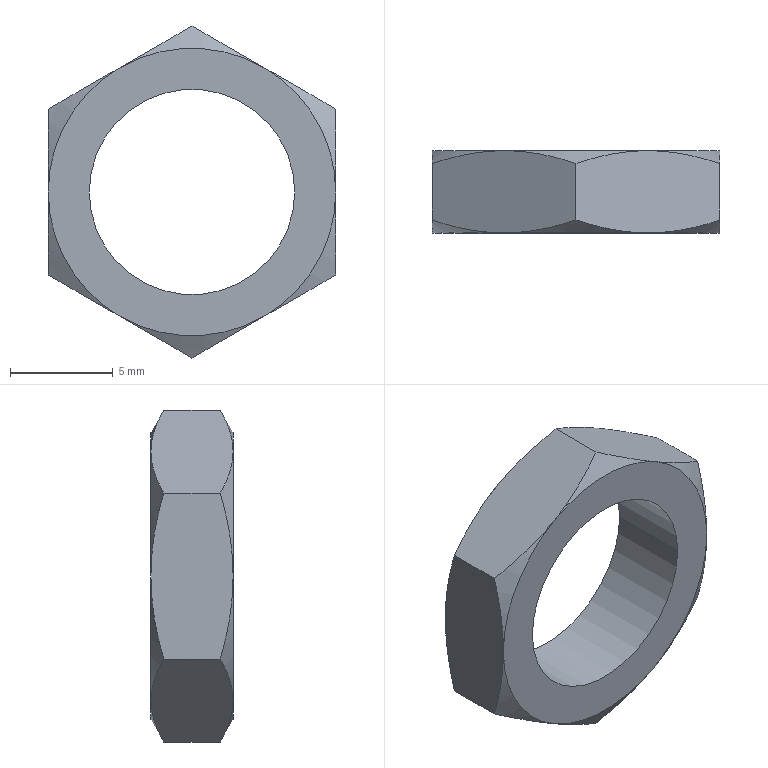Component | SolidWorks | ClampingAssembly-1_RB1006-1_RB1006-2-1 | 1 solid | 22 faces | box 14 x 4 x 16.17 mm | volume 359 mm3 | cone 12 | plane 8 | cylinder 2 | commonest cylinder face diameters 10 x2
STEP:
#1=COLOUR_RGB('',0.7922,0.8196,0.9333);
#2=FILL_AREA_STYLE_COLOUR('',#1);
#3=FILL_AREA_STYLE('',(#2));
#4=SURFACE_STYLE_FILL_AREA(#3);
#5=SURFACE_SIDE_STYLE('',(#4));
#6=SURFACE_STYLE_USAGE(.BOTH.,#5);
#7=PRESENTATION_STYLE_ASSIGNMENT((#6));
#8=CARTESIAN_POINT('',(-0.1398,4.726,-1.201));
#9=VERTEX_POINT('',#8);
#10=CARTESIAN_POINT('',(-0.5335,4.726,-1.201));
#11=VERTEX_POINT('',#10);
#12=CARTESIAN_POINT('',(-0.3366,4.726,-1.201));
#13=DIRECTION('',(-0.,1.,-0.));
#14=DIRECTION('',(-1.,0.,0.));
#15=AXIS2_PLACEMENT_3D('',#12,#13,#14);
#16=CIRCLE('',#15,0.1969);
#17=EDGE_CURVE('',#9,#11,#16,.T.);
#18=ORIENTED_EDGE('',*,*,#17,.T.);
#19=CARTESIAN_POINT('',(-0.5335,4.568,-1.201));
#20=VERTEX_POINT('',#19);
#21=CARTESIAN_POINT('',(-0.5335,4.568,-1.201));
#22=DIRECTION('',(0.,-1.,0.));
#23=VECTOR('',#22,39.37);
#24=LINE('',#21,#23);
#25=EDGE_CURVE('',#11,#20,#24,.T.);
#26=ORIENTED_EDGE('',*,*,#25,.T.);
#27=CARTESIAN_POINT('',(-0.1398,4.568,-1.201));
#28=VERTEX_POINT('',#27);
#29=CARTESIAN_POINT('',(-0.3366,4.568,-1.201));
#30=DIRECTION('',(-0.,1.,-0.));
#31=DIRECTION('',(1.,0.,0.));
#32=AXIS2_PLACEMENT_3D('',#29,#30,#31);
#33=CIRCLE('',#32,0.1969);
#34=EDGE_CURVE('',#28,#20,#33,.T.);
#35=ORIENTED_EDGE('',*,*,#34,.F.);
#36=CARTESIAN_POINT('',(-0.1398,4.568,-1.201));
#37=DIRECTION('',(0.,-1.,0.));
#38=VECTOR('',#37,39.37);
#39=LINE('',#36,#38);
#40=EDGE_CURVE('',#9,#28,#39,.T.);
#41=ORIENTED_EDGE('',*,*,#40,.F.);
#42=EDGE_LOOP('',(#18,#26,#35,#41));
#43=FACE_OUTER_BOUND('',#42,.T.);
#44=CARTESIAN_POINT('',(-0.3366,4.568,-1.201));
#45=DIRECTION('',(0.,-1.,0.));
#46=DIRECTION('',(1.,0.,0.));
#47=AXIS2_PLACEMENT_3D('',#44,#45,#46);
#48=CYLINDRICAL_SURFACE('',#47,0.1969);
#49=ADVANCED_FACE('',(#43),#48,.F.);
#50=CARTESIAN_POINT('',(-0.1988,4.568,-1.439));
#51=VERTEX_POINT('',#50);
#52=CARTESIAN_POINT('',(-0.06105,4.568,-1.201));
#53=VERTEX_POINT('',#52);
#54=CARTESIAN_POINT('',(-0.3366,4.568,-1.201));
#55=DIRECTION('',(-0.,-1.,0.));
#56=DIRECTION('',(-1.,0.,0.));
#57=AXIS2_PLACEMENT_3D('',#54,#55,#56);
#58=CIRCLE('',#57,0.2756);
#59=EDGE_CURVE('',#51,#53,#58,.T.);
#60=ORIENTED_EDGE('',*,*,#59,.T.);
#61=CARTESIAN_POINT('',(-0.1988,4.568,-0.9621));
#62=VERTEX_POINT('',#61);
#63=CARTESIAN_POINT('',(-0.3366,4.568,-1.201));
#64=DIRECTION('',(-0.,-1.,0.));
#65=DIRECTION('',(-1.,0.,0.));
#66=AXIS2_PLACEMENT_3D('',#63,#64,#65);
#67=CIRCLE('',#66,0.2756);
#68=EDGE_CURVE('',#53,#62,#67,.T.);
#69=ORIENTED_EDGE('',*,*,#68,.T.);
#70=CARTESIAN_POINT('',(-0.4744,4.568,-0.9621));
#71=VERTEX_POINT('',#70);
#72=CARTESIAN_POINT('',(-0.3366,4.568,-1.201));
#73=DIRECTION('',(0.,-1.,0.));
#74=DIRECTION('',(-1.,0.,0.));
#75=AXIS2_PLACEMENT_3D('',#72,#73,#74);
#76=CIRCLE('',#75,0.2756);
#77=EDGE_CURVE('',#62,#71,#76,.T.);
#78=ORIENTED_EDGE('',*,*,#77,.T.);
#79=CARTESIAN_POINT('',(-0.6122,4.568,-1.201));
#80=VERTEX_POINT('',#79);
#81=CARTESIAN_POINT('',(-0.3366,4.568,-1.201));
#82=DIRECTION('',(-0.,-1.,0.));
#83=DIRECTION('',(-1.,0.,0.));
#84=AXIS2_PLACEMENT_3D('',#81,#82,#83);
#85=CIRCLE('',#84,0.2756);
#86=EDGE_CURVE('',#71,#80,#85,.T.);
#87=ORIENTED_EDGE('',*,*,#86,.T.);
#88=CARTESIAN_POINT('',(-0.4744,4.568,-1.439));
#89=VERTEX_POINT('',#88);
#90=CARTESIAN_POINT('',(-0.3366,4.568,-1.201));
#91=DIRECTION('',(-0.,-1.,0.));
#92=DIRECTION('',(-1.,0.,-0.));
#93=AXIS2_PLACEMENT_3D('',#90,#91,#92);
#94=CIRCLE('',#93,0.2756);
#95=EDGE_CURVE('',#80,#89,#94,.T.);
#96=ORIENTED_EDGE('',*,*,#95,.T.);
#97=CARTESIAN_POINT('',(-0.3366,4.568,-1.201));
#98=DIRECTION('',(0.,-1.,0.));
#99=DIRECTION('',(-1.,0.,0.));
#100=AXIS2_PLACEMENT_3D('',#97,#98,#99);
#101=CIRCLE('',#100,0.2756);
#102=EDGE_CURVE('',#89,#51,#101,.T.);
#103=ORIENTED_EDGE('',*,*,#102,.T.);
#104=EDGE_LOOP('',(#60,#69,#78,#87,#96,#103));
#105=FACE_OUTER_BOUND('',#104,.T.);
#106=ORIENTED_EDGE('',*,*,#34,.T.);
#107=CARTESIAN_POINT('',(-0.3366,4.568,-1.201));
#108=DIRECTION('',(-0.,1.,-0.));
#109=DIRECTION('',(1.,0.,0.));
#110=AXIS2_PLACEMENT_3D('',#107,#108,#109);
#111=CIRCLE('',#110,0.1969);
#112=EDGE_CURVE('',#20,#28,#111,.T.);
#113=ORIENTED_EDGE('',*,*,#112,.T.);
#114=EDGE_LOOP('',(#106,#113));
#115=FACE_BOUND('',#114,.T.);
#116=CARTESIAN_POINT('',(-0.3366,4.568,-0.9646));
#117=DIRECTION('',(0.,-1.,0.));
#118=DIRECTION('',(1.,0.,-0.));
#119=AXIS2_PLACEMENT_3D('',#116,#117,#118);
#120=PLANE('',#119);
#121=ADVANCED_FACE('',(#105,#115),#120,.T.);
#122=CARTESIAN_POINT('',(-0.06105,4.593,-1.042));
#123=VERTEX_POINT('',#122);
#124=CARTESIAN_POINT('',(-0.06105,4.593,-1.042));
#125=CARTESIAN_POINT('',(-0.08356,4.585,-1.029));
#126=CARTESIAN_POINT('',(-0.1063,4.579,-1.016));
#127=CARTESIAN_POINT('',(-0.1521,4.571,-0.9891));
#128=CARTESIAN_POINT('',(-0.1753,4.568,-0.9757));
#129=CARTESIAN_POINT('',(-0.1988,4.568,-0.9621));
#130=B_SPLINE_CURVE_WITH_KNOTS('',3,(#124,#125,#126,#127,#128,#129),.UNSPECIFIED.,.F.,.F.,(4,2,4),(0.,0.002045,0.00409),.UNSPECIFIED.);
#131=EDGE_CURVE('',#123,#62,#130,.T.);
#132=ORIENTED_EDGE('',*,*,#131,.T.);
#133=ORIENTED_EDGE('',*,*,#68,.F.);
#134=CARTESIAN_POINT('',(-0.06105,4.568,-1.201));
#135=CARTESIAN_POINT('',(-0.06105,4.568,-1.174));
#136=CARTESIAN_POINT('',(-0.06105,4.571,-1.147));
#137=CARTESIAN_POINT('',(-0.06105,4.579,-1.094));
#138=CARTESIAN_POINT('',(-0.06105,4.585,-1.068));
#139=CARTESIAN_POINT('',(-0.06105,4.593,-1.042));
#140=B_SPLINE_CURVE_WITH_KNOTS('',3,(#134,#135,#136,#137,#138,#139),.UNSPECIFIED.,.F.,.F.,(4,2,4),(0.,0.002045,0.00409),.UNSPECIFIED.);
#141=EDGE_CURVE('',#53,#123,#140,.T.);
#142=ORIENTED_EDGE('',*,*,#141,.T.);
#143=EDGE_LOOP('',(#132,#133,#142));
#144=FACE_OUTER_BOUND('',#143,.T.);
#145=CARTESIAN_POINT('',(-0.3366,4.593,-1.201));
#146=DIRECTION('',(0.,1.,-0.));
#147=DIRECTION('',(-1.,0.,0.));
#148=AXIS2_PLACEMENT_3D('',#145,#146,#147);
#149=CONICAL_SURFACE('',#148,0.3185,1.047);
#150=ADVANCED_FACE('',(#144),#149,.T.);
#151=CARTESIAN_POINT('',(-0.06105,4.593,-1.36));
#152=VERTEX_POINT('',#151);
#153=CARTESIAN_POINT('',(-0.06105,4.593,-1.36));
#154=CARTESIAN_POINT('',(-0.06105,4.585,-1.334));
#155=CARTESIAN_POINT('',(-0.06105,4.579,-1.308));
#156=CARTESIAN_POINT('',(-0.06105,4.571,-1.255));
#157=CARTESIAN_POINT('',(-0.06105,4.568,-1.228));
#158=CARTESIAN_POINT('',(-0.06105,4.568,-1.201));
#159=B_SPLINE_CURVE_WITH_KNOTS('',3,(#153,#154,#155,#156,#157,#158),.UNSPECIFIED.,.F.,.F.,(4,2,4),(0.,0.002045,0.00409),.UNSPECIFIED.);
#160=EDGE_CURVE('',#152,#53,#159,.T.);
#161=ORIENTED_EDGE('',*,*,#160,.T.);
#162=ORIENTED_EDGE('',*,*,#59,.F.);
#163=CARTESIAN_POINT('',(-0.1988,4.568,-1.439));
#164=CARTESIAN_POINT('',(-0.1753,4.568,-1.426));
#165=CARTESIAN_POINT('',(-0.1521,4.571,-1.412));
#166=CARTESIAN_POINT('',(-0.1063,4.579,-1.386));
#167=CARTESIAN_POINT('',(-0.08356,4.585,-1.373));
#168=CARTESIAN_POINT('',(-0.06105,4.593,-1.36));
#169=B_SPLINE_CURVE_WITH_KNOTS('',3,(#163,#164,#165,#166,#167,#168),.UNSPECIFIED.,.F.,.F.,(4,2,4),(0.,0.002045,0.00409),.UNSPECIFIED.);
#170=EDGE_CURVE('',#51,#152,#169,.T.);
#171=ORIENTED_EDGE('',*,*,#170,.T.);
#172=EDGE_LOOP('',(#161,#162,#171));
#173=FACE_OUTER_BOUND('',#172,.T.);
#174=CARTESIAN_POINT('',(-0.3366,4.593,-1.201));
#175=DIRECTION('',(0.,1.,-0.));
#176=DIRECTION('',(-1.,0.,0.));
#177=AXIS2_PLACEMENT_3D('',#174,#175,#176);
#178=CONICAL_SURFACE('',#177,0.3185,1.047);
#179=ADVANCED_FACE('',(#173),#178,.T.);
#180=CARTESIAN_POINT('',(-0.3366,4.593,-1.519));
#181=VERTEX_POINT('',#180);
#182=CARTESIAN_POINT('',(-0.3366,4.593,-1.519));
#183=CARTESIAN_POINT('',(-0.3141,4.585,-1.506));
#184=CARTESIAN_POINT('',(-0.2914,4.579,-1.493));
#185=CARTESIAN_POINT('',(-0.2456,4.571,-1.466));
#186=CARTESIAN_POINT('',(-0.2224,4.568,-1.453));
#187=CARTESIAN_POINT('',(-0.1988,4.568,-1.439));
#188=B_SPLINE_CURVE_WITH_KNOTS('',3,(#182,#183,#184,#185,#186,#187),.UNSPECIFIED.,.F.,.F.,(4,2,4),(0.,0.002045,0.00409),.UNSPECIFIED.);
#189=EDGE_CURVE('',#181,#51,#188,.T.);
#190=ORIENTED_EDGE('',*,*,#189,.T.);
#191=ORIENTED_EDGE('',*,*,#102,.F.);
#192=CARTESIAN_POINT('',(-0.4744,4.568,-1.439));
#193=CARTESIAN_POINT('',(-0.4509,4.568,-1.453));
#194=CARTESIAN_POINT('',(-0.4277,4.571,-1.466));
#195=CARTESIAN_POINT('',(-0.3818,4.579,-1.493));
#196=CARTESIAN_POINT('',(-0.3592,4.585,-1.506));
#197=CARTESIAN_POINT('',(-0.3366,4.593,-1.519));
#198=B_SPLINE_CURVE_WITH_KNOTS('',3,(#192,#193,#194,#195,#196,#197),.UNSPECIFIED.,.F.,.F.,(4,2,4),(0.,0.002045,0.00409),.UNSPECIFIED.);
#199=EDGE_CURVE('',#89,#181,#198,.T.);
#200=ORIENTED_EDGE('',*,*,#199,.T.);
#201=EDGE_LOOP('',(#190,#191,#200));
#202=FACE_OUTER_BOUND('',#201,.T.);
#203=CARTESIAN_POINT('',(-0.3366,4.593,-1.201));
#204=DIRECTION('',(-0.,1.,-0.));
#205=DIRECTION('',(-1.,0.,0.));
#206=AXIS2_PLACEMENT_3D('',#203,#204,#205);
#207=CONICAL_SURFACE('',#206,0.3185,1.047);
#208=ADVANCED_FACE('',(#202),#207,.T.);
#209=ORIENTED_EDGE('',*,*,#95,.F.);
#210=CARTESIAN_POINT('',(-0.6122,4.593,-1.36));
#211=VERTEX_POINT('',#210);
#212=CARTESIAN_POINT('',(-0.6122,4.568,-1.201));
#213=CARTESIAN_POINT('',(-0.6122,4.568,-1.228));
#214=CARTESIAN_POINT('',(-0.6122,4.571,-1.255));
#215=CARTESIAN_POINT('',(-0.6122,4.579,-1.308));
#216=CARTESIAN_POINT('',(-0.6122,4.585,-1.334));
#217=CARTESIAN_POINT('',(-0.6122,4.593,-1.36));
#218=B_SPLINE_CURVE_WITH_KNOTS('',3,(#212,#213,#214,#215,#216,#217),.UNSPECIFIED.,.F.,.F.,(4,2,4),(0.,0.002045,0.00409),.UNSPECIFIED.);
#219=EDGE_CURVE('',#80,#211,#218,.T.);
#220=ORIENTED_EDGE('',*,*,#219,.T.);
#221=CARTESIAN_POINT('',(-0.6122,4.593,-1.36));
#222=CARTESIAN_POINT('',(-0.5897,4.585,-1.373));
#223=CARTESIAN_POINT('',(-0.567,4.579,-1.386));
#224=CARTESIAN_POINT('',(-0.5212,4.571,-1.412));
#225=CARTESIAN_POINT('',(-0.498,4.568,-1.426));
#226=CARTESIAN_POINT('',(-0.4744,4.568,-1.439));
#227=B_SPLINE_CURVE_WITH_KNOTS('',3,(#221,#222,#223,#224,#225,#226),.UNSPECIFIED.,.F.,.F.,(4,2,4),(0.,0.002045,0.00409),.UNSPECIFIED.);
#228=EDGE_CURVE('',#211,#89,#227,.T.);
#229=ORIENTED_EDGE('',*,*,#228,.T.);
#230=EDGE_LOOP('',(#209,#220,#229));
#231=FACE_OUTER_BOUND('',#230,.T.);
#232=CARTESIAN_POINT('',(-0.3366,4.593,-1.201));
#233=DIRECTION('',(0.,1.,-0.));
#234=DIRECTION('',(-1.,0.,0.));
#235=AXIS2_PLACEMENT_3D('',#232,#233,#234);
#236=CONICAL_SURFACE('',#235,0.3185,1.047);
#237=ADVANCED_FACE('',(#231),#236,.T.);
#238=ORIENTED_EDGE('',*,*,#86,.F.);
#239=CARTESIAN_POINT('',(-0.6122,4.593,-1.042));
#240=VERTEX_POINT('',#239);
#241=CARTESIAN_POINT('',(-0.4744,4.568,-0.9621));
#242=CARTESIAN_POINT('',(-0.498,4.568,-0.9757));
#243=CARTESIAN_POINT('',(-0.5212,4.571,-0.9891));
#244=CARTESIAN_POINT('',(-0.567,4.579,-1.016));
#245=CARTESIAN_POINT('',(-0.5897,4.585,-1.029));
#246=CARTESIAN_POINT('',(-0.6122,4.593,-1.042));
#247=B_SPLINE_CURVE_WITH_KNOTS('',3,(#241,#242,#243,#244,#245,#246),.UNSPECIFIED.,.F.,.F.,(4,2,4),(0.,0.002045,0.00409),.UNSPECIFIED.);
#248=EDGE_CURVE('',#71,#240,#247,.T.);
#249=ORIENTED_EDGE('',*,*,#248,.T.);
#250=CARTESIAN_POINT('',(-0.6122,4.593,-1.042));
#251=CARTESIAN_POINT('',(-0.6122,4.585,-1.068));
#252=CARTESIAN_POINT('',(-0.6122,4.579,-1.094));
#253=CARTESIAN_POINT('',(-0.6122,4.571,-1.147));
#254=CARTESIAN_POINT('',(-0.6122,4.568,-1.174));
#255=CARTESIAN_POINT('',(-0.6122,4.568,-1.201));
#256=B_SPLINE_CURVE_WITH_KNOTS('',3,(#250,#251,#252,#253,#254,#255),.UNSPECIFIED.,.F.,.F.,(4,2,4),(0.,0.002045,0.00409),.UNSPECIFIED.);
#257=EDGE_CURVE('',#240,#80,#256,.T.);
#258=ORIENTED_EDGE('',*,*,#257,.T.);
#259=EDGE_LOOP('',(#238,#249,#258));
#260=FACE_OUTER_BOUND('',#259,.T.);
#261=CARTESIAN_POINT('',(-0.3366,4.593,-1.201));
#262=DIRECTION('',(0.,1.,-0.));
#263=DIRECTION('',(-1.,0.,0.));
#264=AXIS2_PLACEMENT_3D('',#261,#262,#263);
#265=CONICAL_SURFACE('',#264,0.3185,1.047);
#266=ADVANCED_FACE('',(#260),#265,.T.);
#267=CARTESIAN_POINT('',(-0.3366,4.593,-0.8826));
#268=VERTEX_POINT('',#267);
#269=CARTESIAN_POINT('',(-0.3366,4.593,-0.8826));
#270=CARTESIAN_POINT('',(-0.3592,4.585,-0.8956));
#271=CARTESIAN_POINT('',(-0.3818,4.579,-0.9087));
#272=CARTESIAN_POINT('',(-0.4277,4.571,-0.9351));
#273=CARTESIAN_POINT('',(-0.4509,4.568,-0.9485));
#274=CARTESIAN_POINT('',(-0.4744,4.568,-0.9621));
#275=B_SPLINE_CURVE_WITH_KNOTS('',3,(#269,#270,#271,#272,#273,#274),.UNSPECIFIED.,.F.,.F.,(4,2,4),(0.,0.002045,0.00409),.UNSPECIFIED.);
#276=EDGE_CURVE('',#268,#71,#275,.T.);
#277=ORIENTED_EDGE('',*,*,#276,.T.);
#278=ORIENTED_EDGE('',*,*,#77,.F.);
#279=CARTESIAN_POINT('',(-0.1988,4.568,-0.9621));
#280=CARTESIAN_POINT('',(-0.2224,4.568,-0.9485));
#281=CARTESIAN_POINT('',(-0.2456,4.571,-0.9351));
#282=CARTESIAN_POINT('',(-0.2914,4.579,-0.9087));
#283=CARTESIAN_POINT('',(-0.3141,4.585,-0.8956));
#284=CARTESIAN_POINT('',(-0.3366,4.593,-0.8826));
#285=B_SPLINE_CURVE_WITH_KNOTS('',3,(#279,#280,#281,#282,#283,#284),.UNSPECIFIED.,.F.,.F.,(4,2,4),(0.,0.002045,0.00409),.UNSPECIFIED.);
#286=EDGE_CURVE('',#62,#268,#285,.T.);
#287=ORIENTED_EDGE('',*,*,#286,.T.);
#288=EDGE_LOOP('',(#277,#278,#287));
#289=FACE_OUTER_BOUND('',#288,.T.);
#290=CARTESIAN_POINT('',(-0.3366,4.593,-1.201));
#291=DIRECTION('',(-0.,1.,-0.));
#292=DIRECTION('',(-1.,0.,0.));
#293=AXIS2_PLACEMENT_3D('',#290,#291,#292);
#294=CONICAL_SURFACE('',#293,0.3185,1.047);
#295=ADVANCED_FACE('',(#289),#294,.T.);
#296=CARTESIAN_POINT('',(-0.3366,4.701,-0.8826));
#297=VERTEX_POINT('',#296);
#298=CARTESIAN_POINT('',(-0.3366,4.568,-0.8826));
#299=DIRECTION('',(-0.,1.,-0.));
#300=VECTOR('',#299,39.37);
#301=LINE('',#298,#300);
#302=EDGE_CURVE('',#268,#297,#301,.T.);
#303=ORIENTED_EDGE('',*,*,#302,.F.);
#304=ORIENTED_EDGE('',*,*,#286,.F.);
#305=ORIENTED_EDGE('',*,*,#131,.F.);
#306=CARTESIAN_POINT('',(-0.06105,4.701,-1.042));
#307=VERTEX_POINT('',#306);
#308=CARTESIAN_POINT('',(-0.06105,4.568,-1.042));
#309=DIRECTION('',(0.,-1.,0.));
#310=VECTOR('',#309,39.37);
#311=LINE('',#308,#310);
#312=EDGE_CURVE('',#307,#123,#311,.T.);
#313=ORIENTED_EDGE('',*,*,#312,.F.);
#314=CARTESIAN_POINT('',(-0.1988,4.726,-0.9621));
#315=VERTEX_POINT('',#314);
#316=CARTESIAN_POINT('',(-0.1988,4.726,-0.9621));
#317=CARTESIAN_POINT('',(-0.1753,4.726,-0.9757));
#318=CARTESIAN_POINT('',(-0.1521,4.723,-0.9891));
#319=CARTESIAN_POINT('',(-0.1063,4.715,-1.016));
#320=CARTESIAN_POINT('',(-0.08356,4.709,-1.029));
#321=CARTESIAN_POINT('',(-0.06105,4.701,-1.042));
#322=B_SPLINE_CURVE_WITH_KNOTS('',3,(#316,#317,#318,#319,#320,#321),.UNSPECIFIED.,.F.,.F.,(4,2,4),(0.,0.002045,0.00409),.UNSPECIFIED.);
#323=EDGE_CURVE('',#315,#307,#322,.T.);
#324=ORIENTED_EDGE('',*,*,#323,.F.);
#325=CARTESIAN_POINT('',(-0.3366,4.701,-0.8826));
#326=CARTESIAN_POINT('',(-0.3141,4.709,-0.8956));
#327=CARTESIAN_POINT('',(-0.2914,4.715,-0.9087));
#328=CARTESIAN_POINT('',(-0.2456,4.723,-0.9351));
#329=CARTESIAN_POINT('',(-0.2224,4.726,-0.9485));
#330=CARTESIAN_POINT('',(-0.1988,4.726,-0.9621));
#331=B_SPLINE_CURVE_WITH_KNOTS('',3,(#325,#326,#327,#328,#329,#330),.UNSPECIFIED.,.F.,.F.,(4,2,4),(0.,0.002045,0.00409),.UNSPECIFIED.);
#332=EDGE_CURVE('',#297,#315,#331,.T.);
#333=ORIENTED_EDGE('',*,*,#332,.F.);
#334=EDGE_LOOP('',(#303,#304,#305,#313,#324,#333));
#335=FACE_OUTER_BOUND('',#334,.T.);
#336=CARTESIAN_POINT('',(-0.3366,4.568,-0.8826));
#337=DIRECTION('',(-0.5,-0.,-0.866));
#338=DIRECTION('',(-0.866,-0.,0.5));
#339=AXIS2_PLACEMENT_3D('',#336,#337,#338);
#340=PLANE('',#339);
#341=ADVANCED_FACE('',(#335),#340,.F.);
#342=CARTESIAN_POINT('',(-0.06105,4.726,-1.201));
#343=VERTEX_POINT('',#342);
#344=CARTESIAN_POINT('',(-0.06105,4.701,-1.042));
#345=CARTESIAN_POINT('',(-0.06105,4.709,-1.068));
#346=CARTESIAN_POINT('',(-0.06105,4.715,-1.094));
#347=CARTESIAN_POINT('',(-0.06105,4.723,-1.147));
#348=CARTESIAN_POINT('',(-0.06105,4.726,-1.174));
#349=CARTESIAN_POINT('',(-0.06105,4.726,-1.201));
#350=B_SPLINE_CURVE_WITH_KNOTS('',3,(#344,#345,#346,#347,#348,#349),.UNSPECIFIED.,.F.,.F.,(4,2,4),(0.,0.002045,0.00409),.UNSPECIFIED.);
#351=EDGE_CURVE('',#307,#343,#350,.T.);
#352=ORIENTED_EDGE('',*,*,#351,.F.);
#353=ORIENTED_EDGE('',*,*,#312,.T.);
#354=ORIENTED_EDGE('',*,*,#141,.F.);
#355=ORIENTED_EDGE('',*,*,#160,.F.);
#356=CARTESIAN_POINT('',(-0.06105,4.701,-1.36));
#357=VERTEX_POINT('',#356);
#358=CARTESIAN_POINT('',(-0.06105,4.568,-1.36));
#359=DIRECTION('',(0.,-1.,0.));
#360=VECTOR('',#359,39.37);
#361=LINE('',#358,#360);
#362=EDGE_CURVE('',#357,#152,#361,.T.);
#363=ORIENTED_EDGE('',*,*,#362,.F.);
#364=CARTESIAN_POINT('',(-0.06105,4.726,-1.201));
#365=CARTESIAN_POINT('',(-0.06105,4.726,-1.228));
#366=CARTESIAN_POINT('',(-0.06105,4.723,-1.255));
#367=CARTESIAN_POINT('',(-0.06105,4.715,-1.308));
#368=CARTESIAN_POINT('',(-0.06105,4.709,-1.334));
#369=CARTESIAN_POINT('',(-0.06105,4.701,-1.36));
#370=B_SPLINE_CURVE_WITH_KNOTS('',3,(#364,#365,#366,#367,#368,#369),.UNSPECIFIED.,.F.,.F.,(4,2,4),(0.,0.002045,0.00409),.UNSPECIFIED.);
#371=EDGE_CURVE('',#343,#357,#370,.T.);
#372=ORIENTED_EDGE('',*,*,#371,.F.);
#373=EDGE_LOOP('',(#352,#353,#354,#355,#363,#372));
#374=FACE_OUTER_BOUND('',#373,.T.);
#375=CARTESIAN_POINT('',(-0.06105,4.568,-1.042));
#376=DIRECTION('',(-1.,-0.,0.));
#377=DIRECTION('',(0.,-1.,0.));
#378=AXIS2_PLACEMENT_3D('',#375,#376,#377);
#379=PLANE('',#378);
#380=ADVANCED_FACE('',(#374),#379,.F.);
#381=CARTESIAN_POINT('',(-0.1988,4.726,-1.439));
#382=VERTEX_POINT('',#381);
#383=CARTESIAN_POINT('',(-0.06105,4.701,-1.36));
#384=CARTESIAN_POINT('',(-0.08356,4.709,-1.373));
#385=CARTESIAN_POINT('',(-0.1063,4.715,-1.386));
#386=CARTESIAN_POINT('',(-0.1521,4.723,-1.412));
#387=CARTESIAN_POINT('',(-0.1753,4.726,-1.426));
#388=CARTESIAN_POINT('',(-0.1988,4.726,-1.439));
#389=B_SPLINE_CURVE_WITH_KNOTS('',3,(#383,#384,#385,#386,#387,#388),.UNSPECIFIED.,.F.,.F.,(4,2,4),(0.,0.002045,0.00409),.UNSPECIFIED.);
#390=EDGE_CURVE('',#357,#382,#389,.T.);
#391=ORIENTED_EDGE('',*,*,#390,.F.);
#392=ORIENTED_EDGE('',*,*,#362,.T.);
#393=ORIENTED_EDGE('',*,*,#170,.F.);
#394=ORIENTED_EDGE('',*,*,#189,.F.);
#395=CARTESIAN_POINT('',(-0.3366,4.701,-1.519));
#396=VERTEX_POINT('',#395);
#397=CARTESIAN_POINT('',(-0.3366,4.568,-1.519));
#398=DIRECTION('',(0.,-1.,0.));
#399=VECTOR('',#398,39.37);
#400=LINE('',#397,#399);
#401=EDGE_CURVE('',#396,#181,#400,.T.);
#402=ORIENTED_EDGE('',*,*,#401,.F.);
#403=CARTESIAN_POINT('',(-0.1988,4.726,-1.439));
#404=CARTESIAN_POINT('',(-0.2224,4.726,-1.453));
#405=CARTESIAN_POINT('',(-0.2456,4.723,-1.466));
#406=CARTESIAN_POINT('',(-0.2914,4.715,-1.493));
#407=CARTESIAN_POINT('',(-0.3141,4.709,-1.506));
#408=CARTESIAN_POINT('',(-0.3366,4.701,-1.519));
#409=B_SPLINE_CURVE_WITH_KNOTS('',3,(#403,#404,#405,#406,#407,#408),.UNSPECIFIED.,.F.,.F.,(4,2,4),(0.,0.002045,0.00409),.UNSPECIFIED.);
#410=EDGE_CURVE('',#382,#396,#409,.T.);
#411=ORIENTED_EDGE('',*,*,#410,.F.);
#412=EDGE_LOOP('',(#391,#392,#393,#394,#402,#411));
#413=FACE_OUTER_BOUND('',#412,.T.);
#414=CARTESIAN_POINT('',(-0.06105,4.568,-1.36));
#415=DIRECTION('',(-0.5,0.,0.866));
#416=DIRECTION('',(0.866,0.,0.5));
#417=AXIS2_PLACEMENT_3D('',#414,#415,#416);
#418=PLANE('',#417);
#419=ADVANCED_FACE('',(#413),#418,.F.);
#420=CARTESIAN_POINT('',(-0.4744,4.726,-1.439));
#421=VERTEX_POINT('',#420);
#422=CARTESIAN_POINT('',(-0.3366,4.701,-1.519));
#423=CARTESIAN_POINT('',(-0.3592,4.709,-1.506));
#424=CARTESIAN_POINT('',(-0.3818,4.715,-1.493));
#425=CARTESIAN_POINT('',(-0.4277,4.723,-1.466));
#426=CARTESIAN_POINT('',(-0.4509,4.726,-1.453));
#427=CARTESIAN_POINT('',(-0.4744,4.726,-1.439));
#428=B_SPLINE_CURVE_WITH_KNOTS('',3,(#422,#423,#424,#425,#426,#427),.UNSPECIFIED.,.F.,.F.,(4,2,4),(0.,0.002045,0.00409),.UNSPECIFIED.);
#429=EDGE_CURVE('',#396,#421,#428,.T.);
#430=ORIENTED_EDGE('',*,*,#429,.F.);
#431=ORIENTED_EDGE('',*,*,#401,.T.);
#432=ORIENTED_EDGE('',*,*,#199,.F.);
#433=ORIENTED_EDGE('',*,*,#228,.F.);
#434=CARTESIAN_POINT('',(-0.6122,4.701,-1.36));
#435=VERTEX_POINT('',#434);
#436=CARTESIAN_POINT('',(-0.6122,4.568,-1.36));
#437=DIRECTION('',(0.,-1.,0.));
#438=VECTOR('',#437,39.37);
#439=LINE('',#436,#438);
#440=EDGE_CURVE('',#435,#211,#439,.T.);
#441=ORIENTED_EDGE('',*,*,#440,.F.);
#442=CARTESIAN_POINT('',(-0.4744,4.726,-1.439));
#443=CARTESIAN_POINT('',(-0.498,4.726,-1.426));
#444=CARTESIAN_POINT('',(-0.5212,4.723,-1.412));
#445=CARTESIAN_POINT('',(-0.567,4.715,-1.386));
#446=CARTESIAN_POINT('',(-0.5897,4.709,-1.373));
#447=CARTESIAN_POINT('',(-0.6122,4.701,-1.36));
#448=B_SPLINE_CURVE_WITH_KNOTS('',3,(#442,#443,#444,#445,#446,#447),.UNSPECIFIED.,.F.,.F.,(4,2,4),(0.,0.002045,0.00409),.UNSPECIFIED.);
#449=EDGE_CURVE('',#421,#435,#448,.T.);
#450=ORIENTED_EDGE('',*,*,#449,.F.);
#451=EDGE_LOOP('',(#430,#431,#432,#433,#441,#450));
#452=FACE_OUTER_BOUND('',#451,.T.);
#453=CARTESIAN_POINT('',(-0.3366,4.568,-1.519));
#454=DIRECTION('',(0.5,0.,0.866));
#455=DIRECTION('',(0.866,0.,-0.5));
#456=AXIS2_PLACEMENT_3D('',#453,#454,#455);
#457=PLANE('',#456);
#458=ADVANCED_FACE('',(#452),#457,.F.);
#459=ORIENTED_EDGE('',*,*,#440,.T.);
#460=ORIENTED_EDGE('',*,*,#219,.F.);
#461=ORIENTED_EDGE('',*,*,#257,.F.);
#462=CARTESIAN_POINT('',(-0.6122,4.701,-1.042));
#463=VERTEX_POINT('',#462);
#464=CARTESIAN_POINT('',(-0.6122,4.568,-1.042));
#465=DIRECTION('',(0.,-1.,0.));
#466=VECTOR('',#465,39.37);
#467=LINE('',#464,#466);
#468=EDGE_CURVE('',#463,#240,#467,.T.);
#469=ORIENTED_EDGE('',*,*,#468,.F.);
#470=CARTESIAN_POINT('',(-0.6122,4.726,-1.201));
#471=VERTEX_POINT('',#470);
#472=CARTESIAN_POINT('',(-0.6122,4.726,-1.201));
#473=CARTESIAN_POINT('',(-0.6122,4.726,-1.174));
#474=CARTESIAN_POINT('',(-0.6122,4.723,-1.147));
#475=CARTESIAN_POINT('',(-0.6122,4.715,-1.094));
#476=CARTESIAN_POINT('',(-0.6122,4.709,-1.068));
#477=CARTESIAN_POINT('',(-0.6122,4.701,-1.042));
#478=B_SPLINE_CURVE_WITH_KNOTS('',3,(#472,#473,#474,#475,#476,#477),.UNSPECIFIED.,.F.,.F.,(4,2,4),(0.,0.002045,0.00409),.UNSPECIFIED.);
#479=EDGE_CURVE('',#471,#463,#478,.T.);
#480=ORIENTED_EDGE('',*,*,#479,.F.);
#481=CARTESIAN_POINT('',(-0.6122,4.701,-1.36));
#482=CARTESIAN_POINT('',(-0.6122,4.709,-1.334));
#483=CARTESIAN_POINT('',(-0.6122,4.715,-1.308));
#484=CARTESIAN_POINT('',(-0.6122,4.723,-1.255));
#485=CARTESIAN_POINT('',(-0.6122,4.726,-1.228));
#486=CARTESIAN_POINT('',(-0.6122,4.726,-1.201));
#487=B_SPLINE_CURVE_WITH_KNOTS('',3,(#481,#482,#483,#484,#485,#486),.UNSPECIFIED.,.F.,.F.,(4,2,4),(0.,0.002045,0.00409),.UNSPECIFIED.);
#488=EDGE_CURVE('',#435,#471,#487,.T.);
#489=ORIENTED_EDGE('',*,*,#488,.F.);
#490=EDGE_LOOP('',(#459,#460,#461,#469,#480,#489));
#491=FACE_OUTER_BOUND('',#490,.T.);
#492=CARTESIAN_POINT('',(-0.6122,4.568,-1.36));
#493=DIRECTION('',(1.,0.,-0.));
#494=DIRECTION('',(-0.,1.,-0.));
#495=AXIS2_PLACEMENT_3D('',#492,#493,#494);
#496=PLANE('',#495);
#497=ADVANCED_FACE('',(#491),#496,.F.);
#498=ORIENTED_EDGE('',*,*,#468,.T.);
#499=ORIENTED_EDGE('',*,*,#248,.F.);
#500=ORIENTED_EDGE('',*,*,#276,.F.);
#501=ORIENTED_EDGE('',*,*,#302,.T.);
#502=CARTESIAN_POINT('',(-0.4744,4.726,-0.9621));
#503=VERTEX_POINT('',#502);
#504=CARTESIAN_POINT('',(-0.4744,4.726,-0.9621));
#505=CARTESIAN_POINT('',(-0.4509,4.726,-0.9485));
#506=CARTESIAN_POINT('',(-0.4277,4.723,-0.9351));
#507=CARTESIAN_POINT('',(-0.3818,4.715,-0.9087));
#508=CARTESIAN_POINT('',(-0.3592,4.709,-0.8956));
#509=CARTESIAN_POINT('',(-0.3366,4.701,-0.8826));
#510=B_SPLINE_CURVE_WITH_KNOTS('',3,(#504,#505,#506,#507,#508,#509),.UNSPECIFIED.,.F.,.F.,(4,2,4),(0.,0.002045,0.00409),.UNSPECIFIED.);
#511=EDGE_CURVE('',#503,#297,#510,.T.);
#512=ORIENTED_EDGE('',*,*,#511,.F.);
#513=CARTESIAN_POINT('',(-0.6122,4.701,-1.042));
#514=CARTESIAN_POINT('',(-0.5897,4.709,-1.029));
#515=CARTESIAN_POINT('',(-0.567,4.715,-1.016));
#516=CARTESIAN_POINT('',(-0.5212,4.723,-0.9891));
#517=CARTESIAN_POINT('',(-0.498,4.726,-0.9757));
#518=CARTESIAN_POINT('',(-0.4744,4.726,-0.9621));
#519=B_SPLINE_CURVE_WITH_KNOTS('',3,(#513,#514,#515,#516,#517,#518),.UNSPECIFIED.,.F.,.F.,(4,2,4),(0.,0.002045,0.00409),.UNSPECIFIED.);
#520=EDGE_CURVE('',#463,#503,#519,.T.);
#521=ORIENTED_EDGE('',*,*,#520,.F.);
#522=EDGE_LOOP('',(#498,#499,#500,#501,#512,#521));
#523=FACE_OUTER_BOUND('',#522,.T.);
#524=CARTESIAN_POINT('',(-0.6122,4.568,-1.042));
#525=DIRECTION('',(0.5,-0.,-0.866));
#526=DIRECTION('',(-0.866,-0.,-0.5));
#527=AXIS2_PLACEMENT_3D('',#524,#525,#526);
#528=PLANE('',#527);
#529=ADVANCED_FACE('',(#523),#528,.F.);
#530=ORIENTED_EDGE('',*,*,#332,.T.);
#531=CARTESIAN_POINT('',(-0.3366,4.726,-1.201));
#532=DIRECTION('',(0.,-1.,0.));
#533=DIRECTION('',(1.,0.,0.));
#534=AXIS2_PLACEMENT_3D('',#531,#532,#533);
#535=CIRCLE('',#534,0.2756);
#536=EDGE_CURVE('',#315,#503,#535,.T.);
#537=ORIENTED_EDGE('',*,*,#536,.T.);
#538=ORIENTED_EDGE('',*,*,#511,.T.);
#539=EDGE_LOOP('',(#530,#537,#538));
#540=FACE_OUTER_BOUND('',#539,.T.);
#541=CARTESIAN_POINT('',(-0.3366,4.701,-1.201));
#542=DIRECTION('',(0.,-1.,0.));
#543=DIRECTION('',(1.,0.,0.));
#544=AXIS2_PLACEMENT_3D('',#541,#542,#543);
#545=CONICAL_SURFACE('',#544,0.3185,1.047);
#546=ADVANCED_FACE('',(#540),#545,.T.);
#547=ORIENTED_EDGE('',*,*,#351,.T.);
#548=CARTESIAN_POINT('',(-0.3366,4.726,-1.201));
#549=DIRECTION('',(0.,-1.,0.));
#550=DIRECTION('',(1.,0.,0.));
#551=AXIS2_PLACEMENT_3D('',#548,#549,#550);
#552=CIRCLE('',#551,0.2756);
#553=EDGE_CURVE('',#343,#315,#552,.T.);
#554=ORIENTED_EDGE('',*,*,#553,.T.);
#555=ORIENTED_EDGE('',*,*,#323,.T.);
#556=EDGE_LOOP('',(#547,#554,#555));
#557=FACE_OUTER_BOUND('',#556,.T.);
#558=CARTESIAN_POINT('',(-0.3366,4.701,-1.201));
#559=DIRECTION('',(0.,-1.,0.));
#560=DIRECTION('',(1.,0.,0.));
#561=AXIS2_PLACEMENT_3D('',#558,#559,#560);
#562=CONICAL_SURFACE('',#561,0.3185,1.047);
#563=ADVANCED_FACE('',(#557),#562,.T.);
#564=CARTESIAN_POINT('',(-0.3366,4.726,-1.201));
#565=DIRECTION('',(0.,-1.,0.));
#566=DIRECTION('',(1.,0.,0.));
#567=AXIS2_PLACEMENT_3D('',#564,#565,#566);
#568=CIRCLE('',#567,0.2756);
#569=EDGE_CURVE('',#382,#343,#568,.T.);
#570=ORIENTED_EDGE('',*,*,#569,.T.);
#571=ORIENTED_EDGE('',*,*,#371,.T.);
#572=ORIENTED_EDGE('',*,*,#390,.T.);
#573=EDGE_LOOP('',(#570,#571,#572));
#574=FACE_OUTER_BOUND('',#573,.T.);
#575=CARTESIAN_POINT('',(-0.3366,4.701,-1.201));
#576=DIRECTION('',(0.,-1.,0.));
#577=DIRECTION('',(1.,0.,0.));
#578=AXIS2_PLACEMENT_3D('',#575,#576,#577);
#579=CONICAL_SURFACE('',#578,0.3185,1.047);
#580=ADVANCED_FACE('',(#574),#579,.T.);
#581=CARTESIAN_POINT('',(-0.3366,4.726,-1.201));
#582=DIRECTION('',(0.,-1.,0.));
#583=DIRECTION('',(1.,0.,0.));
#584=AXIS2_PLACEMENT_3D('',#581,#582,#583);
#585=CIRCLE('',#584,0.2756);
#586=EDGE_CURVE('',#421,#382,#585,.T.);
#587=ORIENTED_EDGE('',*,*,#586,.T.);
#588=ORIENTED_EDGE('',*,*,#410,.T.);
#589=ORIENTED_EDGE('',*,*,#429,.T.);
#590=EDGE_LOOP('',(#587,#588,#589));
#591=FACE_OUTER_BOUND('',#590,.T.);
#592=CARTESIAN_POINT('',(-0.3366,4.701,-1.201));
#593=DIRECTION('',(0.,-1.,0.));
#594=DIRECTION('',(1.,0.,0.));
#595=AXIS2_PLACEMENT_3D('',#592,#593,#594);
#596=CONICAL_SURFACE('',#595,0.3185,1.047);
#597=ADVANCED_FACE('',(#591),#596,.T.);
#598=CARTESIAN_POINT('',(-0.3366,4.726,-1.201));
#599=DIRECTION('',(0.,-1.,0.));
#600=DIRECTION('',(1.,0.,0.));
#601=AXIS2_PLACEMENT_3D('',#598,#599,#600);
#602=CIRCLE('',#601,0.2756);
#603=EDGE_CURVE('',#471,#421,#602,.T.);
#604=ORIENTED_EDGE('',*,*,#603,.T.);
#605=ORIENTED_EDGE('',*,*,#449,.T.);
#606=ORIENTED_EDGE('',*,*,#488,.T.);
#607=EDGE_LOOP('',(#604,#605,#606));
#608=FACE_OUTER_BOUND('',#607,.T.);
#609=CARTESIAN_POINT('',(-0.3366,4.701,-1.201));
#610=DIRECTION('',(0.,-1.,0.));
#611=DIRECTION('',(1.,0.,0.));
#612=AXIS2_PLACEMENT_3D('',#609,#610,#611);
#613=CONICAL_SURFACE('',#612,0.3185,1.047);
#614=ADVANCED_FACE('',(#608),#613,.T.);
#615=ORIENTED_EDGE('',*,*,#520,.T.);
#616=CARTESIAN_POINT('',(-0.3366,4.726,-1.201));
#617=DIRECTION('',(0.,-1.,0.));
#618=DIRECTION('',(1.,0.,0.));
#619=AXIS2_PLACEMENT_3D('',#616,#617,#618);
#620=CIRCLE('',#619,0.2756);
#621=EDGE_CURVE('',#503,#471,#620,.T.);
#622=ORIENTED_EDGE('',*,*,#621,.T.);
#623=ORIENTED_EDGE('',*,*,#479,.T.);
#624=EDGE_LOOP('',(#615,#622,#623));
#625=FACE_OUTER_BOUND('',#624,.T.);
#626=CARTESIAN_POINT('',(-0.3366,4.701,-1.201));
#627=DIRECTION('',(0.,-1.,0.));
#628=DIRECTION('',(1.,0.,0.));
#629=AXIS2_PLACEMENT_3D('',#626,#627,#628);
#630=CONICAL_SURFACE('',#629,0.3185,1.047);
#631=ADVANCED_FACE('',(#625),#630,.T.);
#632=ORIENTED_EDGE('',*,*,#17,.F.);
#633=CARTESIAN_POINT('',(-0.3366,4.726,-1.201));
#634=DIRECTION('',(-0.,1.,-0.));
#635=DIRECTION('',(-1.,0.,0.));
#636=AXIS2_PLACEMENT_3D('',#633,#634,#635);
#637=CIRCLE('',#636,0.1969);
#638=EDGE_CURVE('',#11,#9,#637,.T.);
#639=ORIENTED_EDGE('',*,*,#638,.F.);
#640=EDGE_LOOP('',(#632,#639));
#641=FACE_BOUND('',#640,.T.);
#642=ORIENTED_EDGE('',*,*,#621,.F.);
#643=ORIENTED_EDGE('',*,*,#536,.F.);
#644=ORIENTED_EDGE('',*,*,#553,.F.);
#645=ORIENTED_EDGE('',*,*,#569,.F.);
#646=ORIENTED_EDGE('',*,*,#586,.F.);
#647=ORIENTED_EDGE('',*,*,#603,.F.);
#648=EDGE_LOOP('',(#642,#643,#644,#645,#646,#647));
#649=FACE_OUTER_BOUND('',#648,.T.);
#650=CARTESIAN_POINT('',(-0.3366,4.726,-0.9646));
#651=DIRECTION('',(-0.,1.,-0.));
#652=DIRECTION('',(-1.,-0.,0.));
#653=AXIS2_PLACEMENT_3D('',#650,#651,#652);
#654=PLANE('',#653);
#655=ADVANCED_FACE('',(#641,#649),#654,.T.);
#656=ORIENTED_EDGE('',*,*,#25,.F.);
#657=ORIENTED_EDGE('',*,*,#638,.T.);
#658=ORIENTED_EDGE('',*,*,#40,.T.);
#659=ORIENTED_EDGE('',*,*,#112,.F.);
#660=EDGE_LOOP('',(#656,#657,#658,#659));
#661=FACE_OUTER_BOUND('',#660,.T.);
#662=CARTESIAN_POINT('',(-0.3366,4.568,-1.201));
#663=DIRECTION('',(0.,-1.,0.));
#664=DIRECTION('',(1.,0.,0.));
#665=AXIS2_PLACEMENT_3D('',#662,#663,#664);
#666=CYLINDRICAL_SURFACE('',#665,0.1969);
#667=ADVANCED_FACE('',(#661),#666,.F.);
#668=CLOSED_SHELL('',(#49,#121,#150,#179,#208,#237,#266,#295,#341,#380,#419,#458,#497,#529,#546,#563,#580,#597,#614,#631,#655,#667));
#669=MANIFOLD_SOLID_BREP('',#668);
#670=STYLED_ITEM('',(#7),#669);
#671=(LENGTH_UNIT()NAMED_UNIT(*)SI_UNIT($,.METRE.));
#672=LENGTH_MEASURE_WITH_UNIT(LENGTH_MEASURE(0.0254),#671);
#673=DIMENSIONAL_EXPONENTS(1.,0.,0.,0.,0.,0.,0.);
#674=(CONVERSION_BASED_UNIT('',#672)LENGTH_UNIT()NAMED_UNIT(#673));
#675=UNCERTAINTY_MEASURE_WITH_UNIT(LENGTH_MEASURE(0.00001),#674,'','');
#676=(NAMED_UNIT(*)PLANE_ANGLE_UNIT()SI_UNIT($,.RADIAN.));
#677=(NAMED_UNIT(*)SI_UNIT($,.STERADIAN.)SOLID_ANGLE_UNIT());
#678=(GEOMETRIC_REPRESENTATION_CONTEXT(3)GLOBAL_UNCERTAINTY_ASSIGNED_CONTEXT((#675))GLOBAL_UNIT_ASSIGNED_CONTEXT((#674,#676,#677))REPRESENTATION_CONTEXT('',''));
#679=MECHANICAL_DESIGN_GEOMETRIC_PRESENTATION_REPRESENTATION('',(#670),#678);
#680=PRESENTATION_LAYER_ASSIGNMENT('','',(#670));
#681=CARTESIAN_POINT('',(0.,0.,0.));
#682=DIRECTION('',(0.,0.,1.));
#683=DIRECTION('',(1.,0.,0.));
#684=AXIS2_PLACEMENT_3D('',#681,#682,#683);
#685=(LENGTH_UNIT()NAMED_UNIT(*)SI_UNIT($,.METRE.));
#686=LENGTH_MEASURE_WITH_UNIT(LENGTH_MEASURE(0.0254),#685);
#687=DIMENSIONAL_EXPONENTS(1.,0.,0.,0.,0.,0.,0.);
#688=(CONVERSION_BASED_UNIT('',#686)LENGTH_UNIT()NAMED_UNIT(#687));
#689=UNCERTAINTY_MEASURE_WITH_UNIT(LENGTH_MEASURE(0.00001),#688,'','');
#690=(NAMED_UNIT(*)PLANE_ANGLE_UNIT()SI_UNIT($,.RADIAN.));
#691=(NAMED_UNIT(*)SI_UNIT($,.STERADIAN.)SOLID_ANGLE_UNIT());
#692=(GEOMETRIC_REPRESENTATION_CONTEXT(3)GLOBAL_UNCERTAINTY_ASSIGNED_CONTEXT((#689))GLOBAL_UNIT_ASSIGNED_CONTEXT((#688,#690,#691))REPRESENTATION_CONTEXT('',''));
#693=ADVANCED_BREP_SHAPE_REPRESENTATION('',(#669,#684),#692);